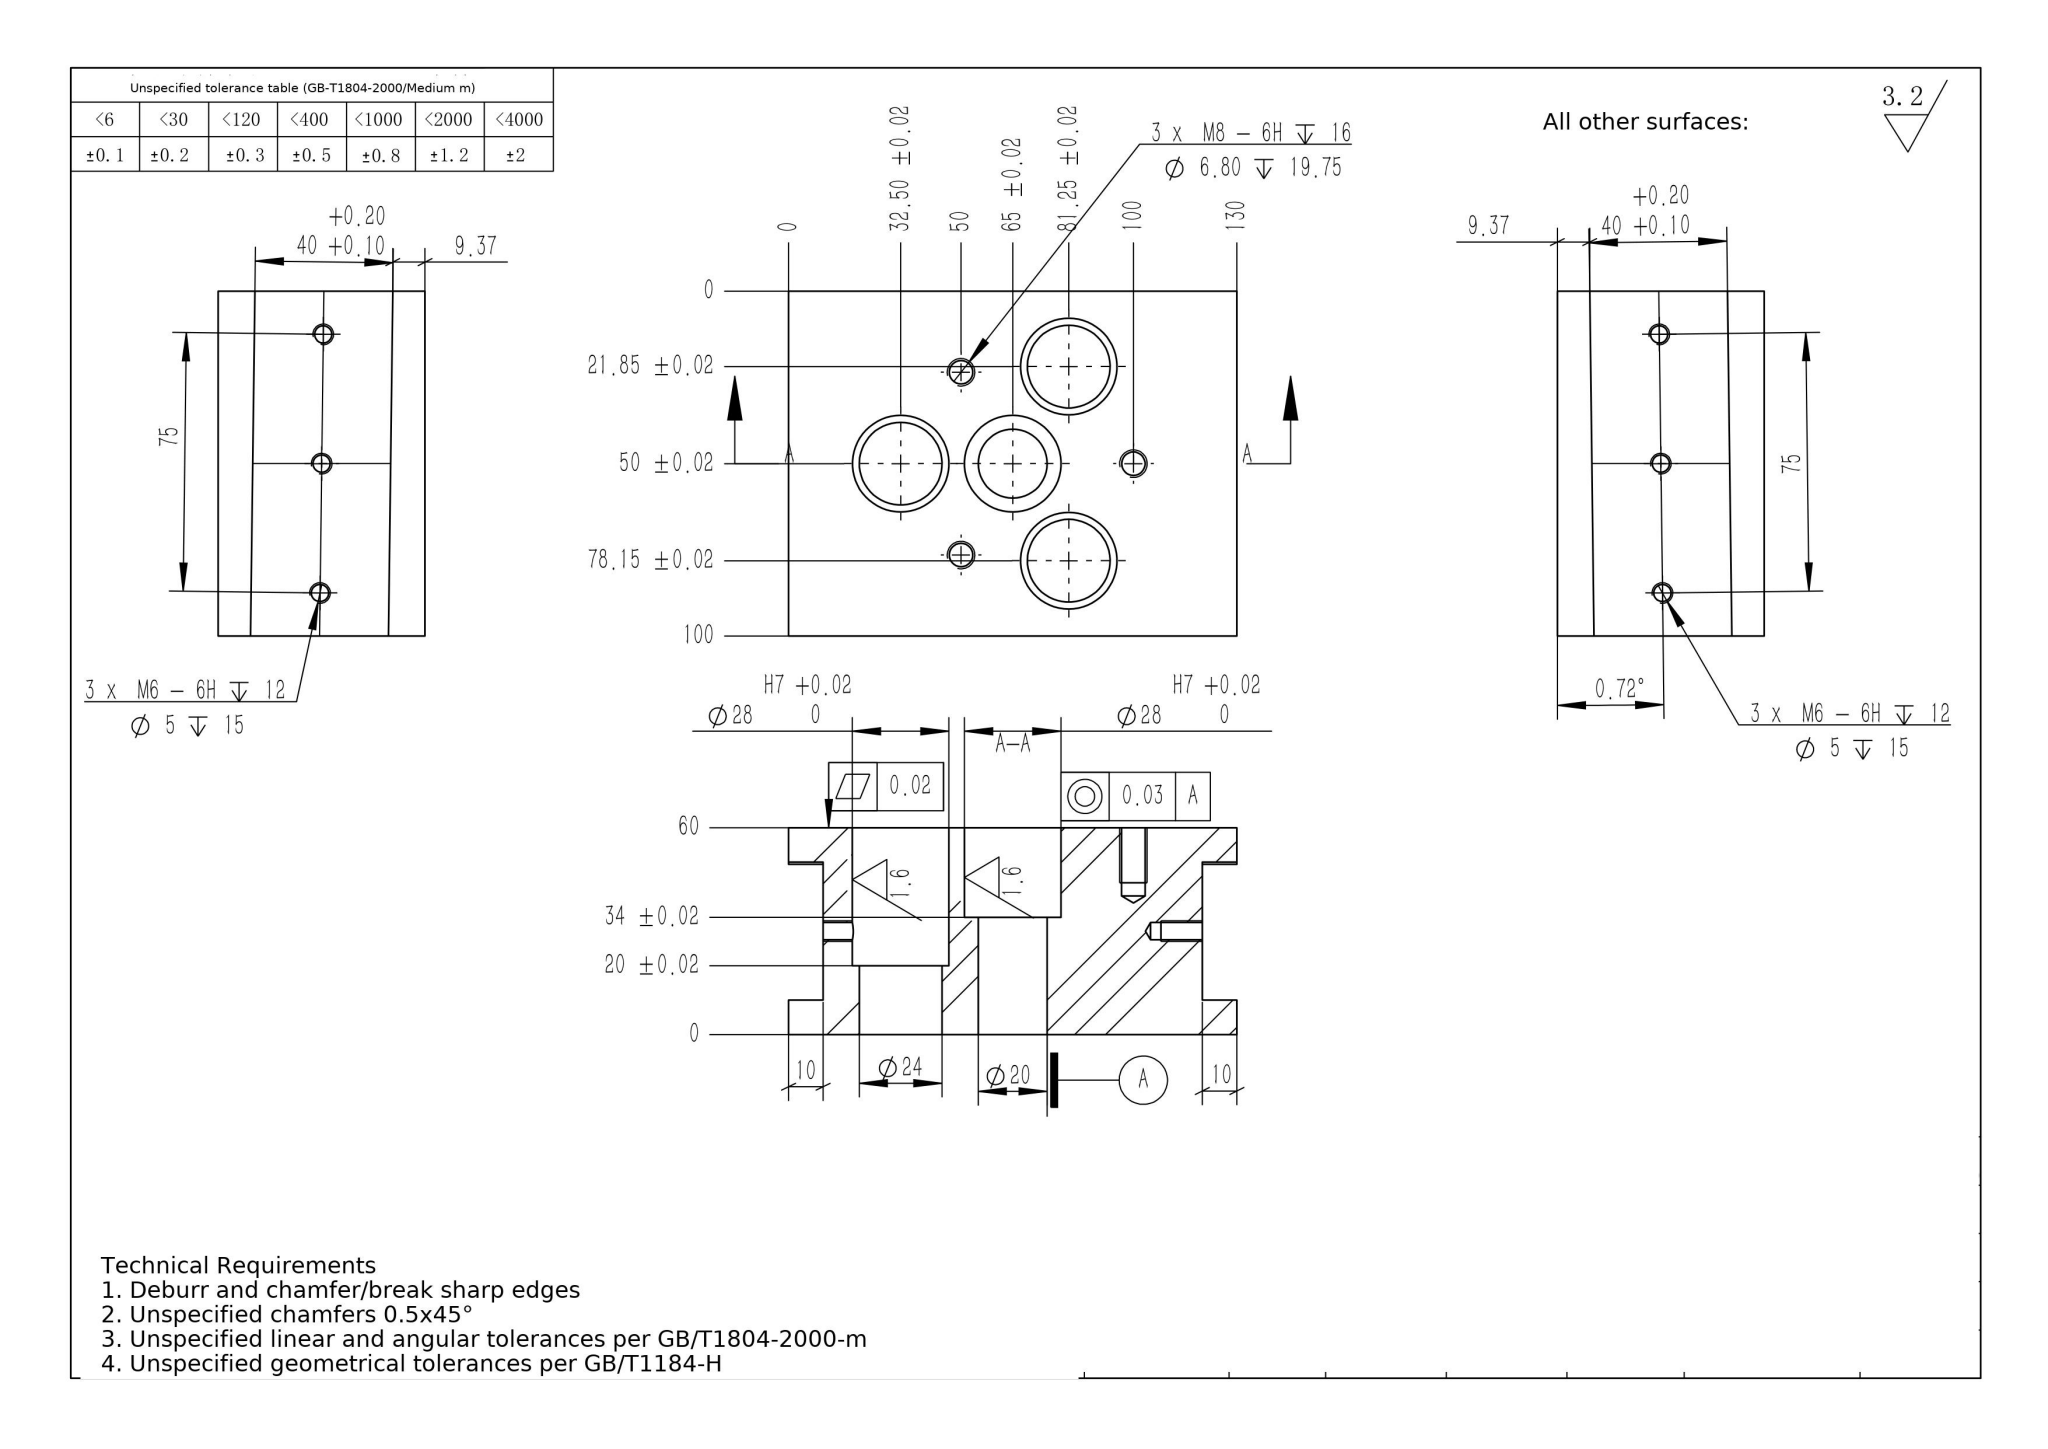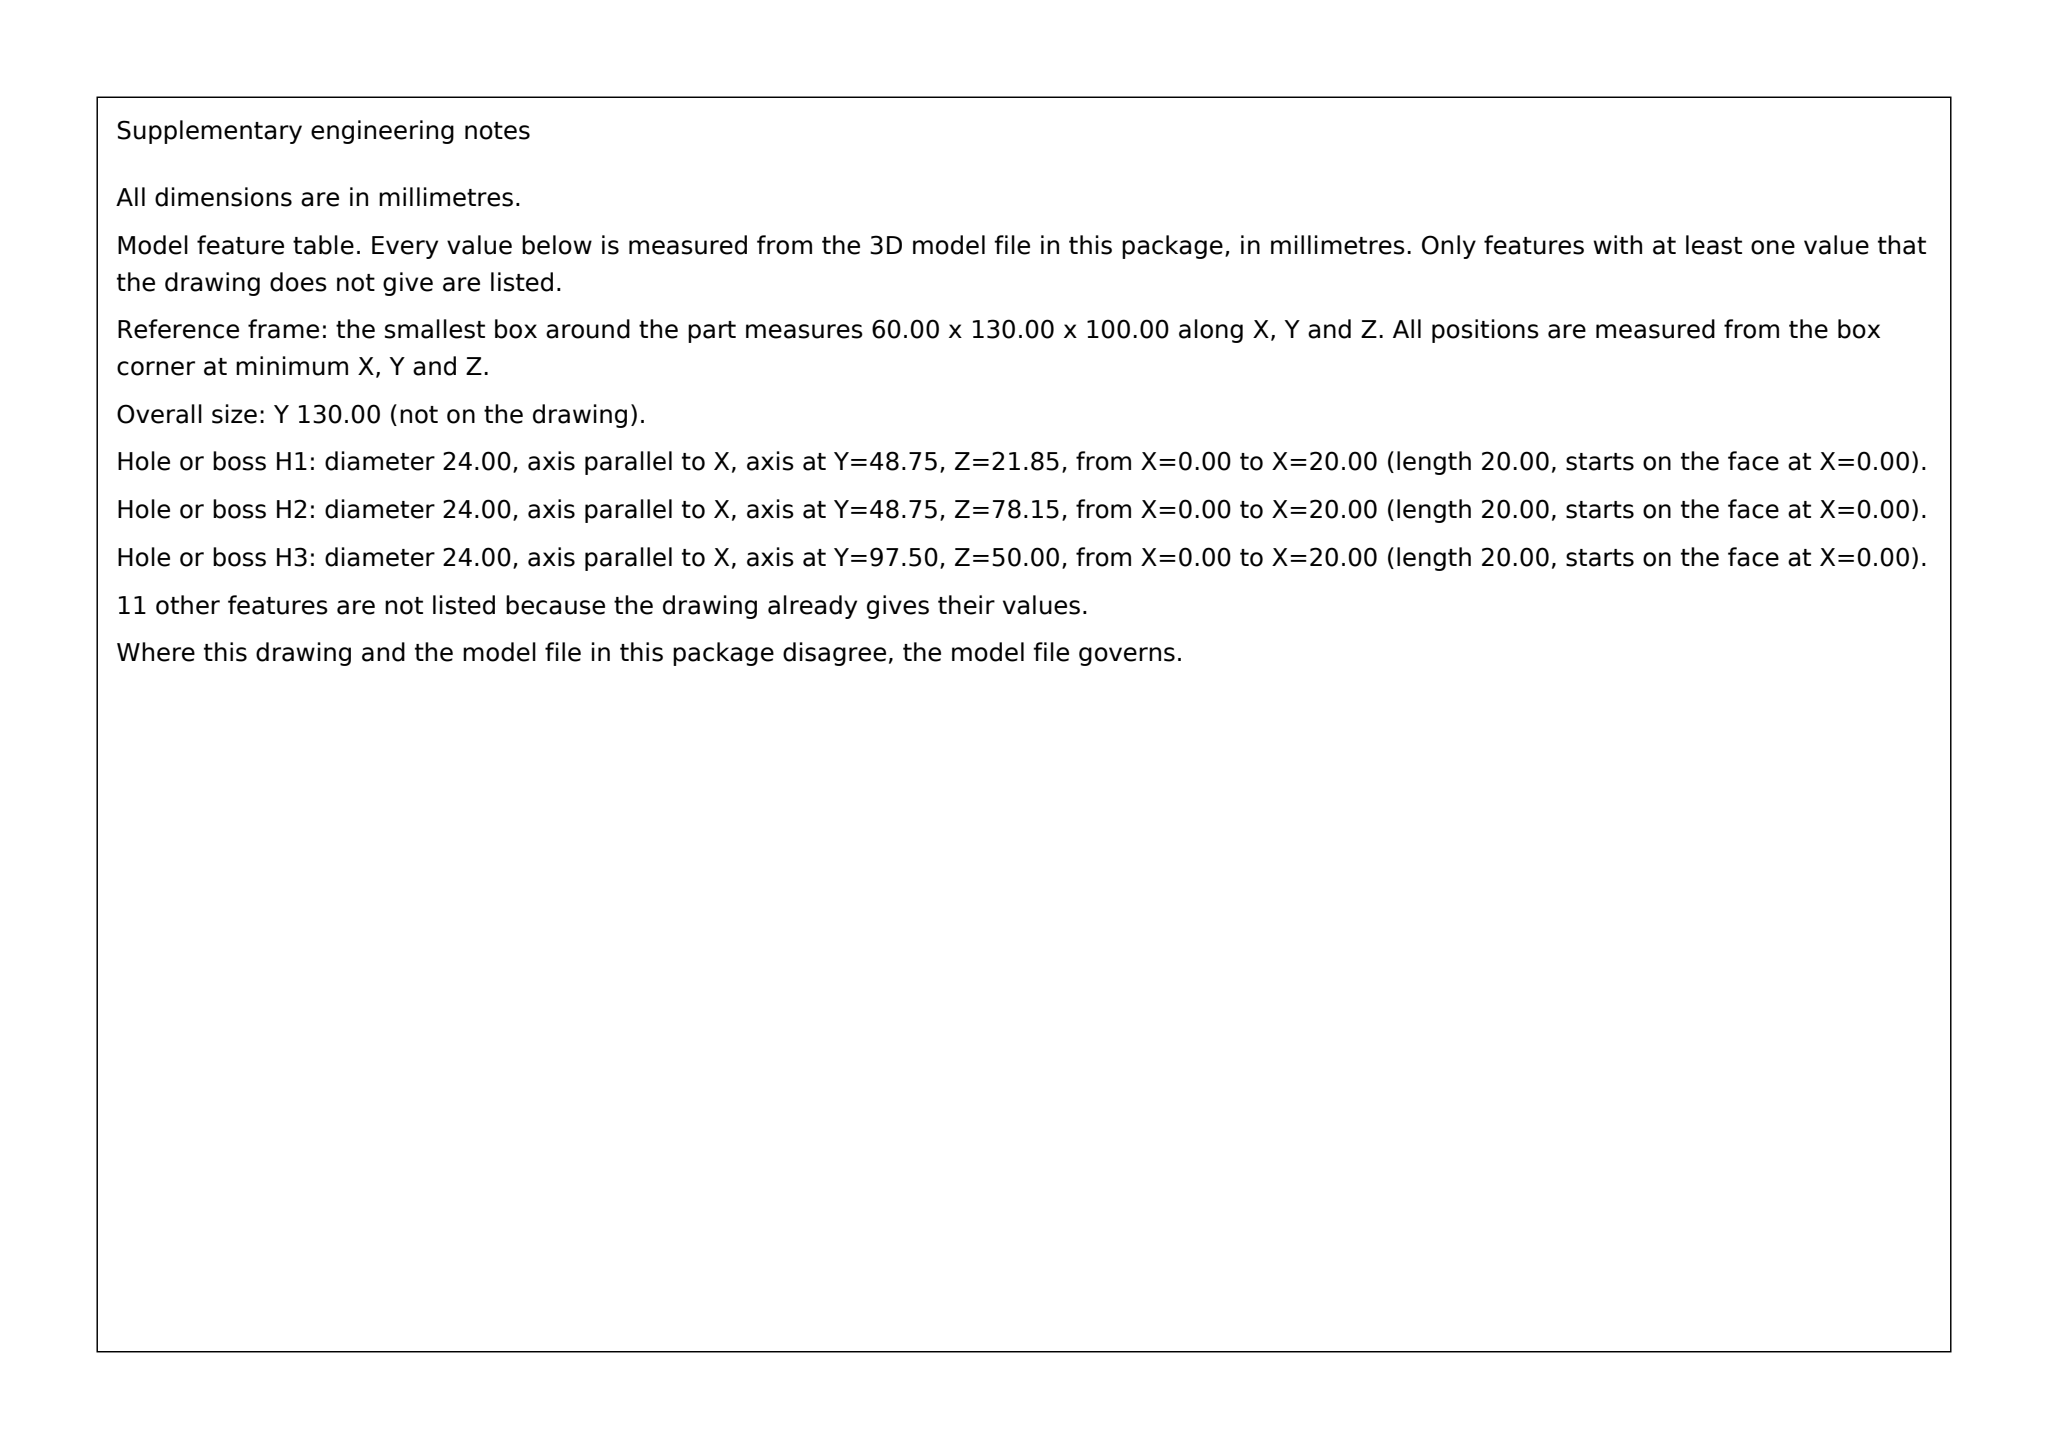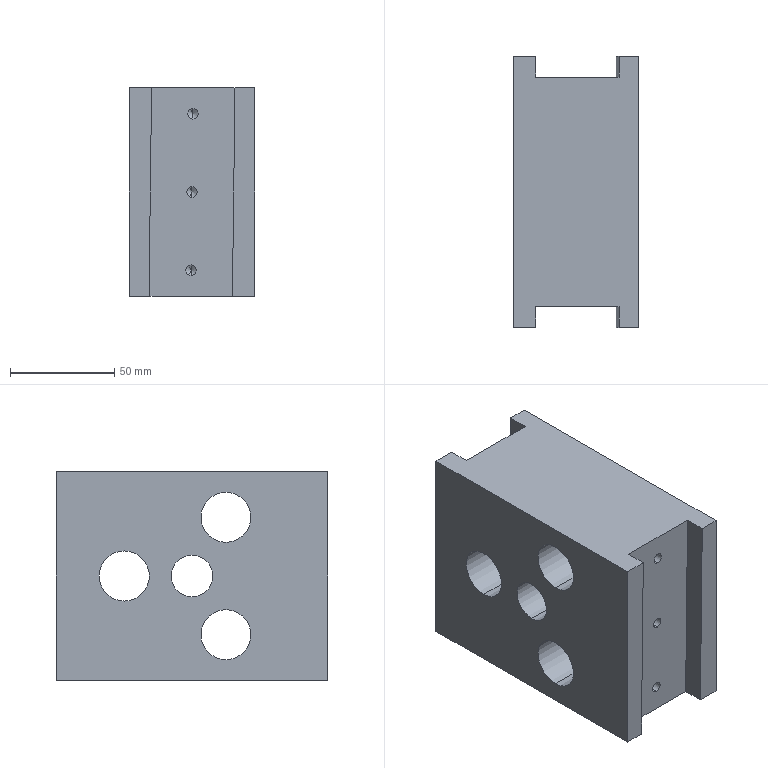Part | SolidWorks | mm | 1 solid | 68 faces | box 60 x 130 x 100 mm | volume 568360 mm3 | cylinder 34 | plane 18 | cone 16 | commonest cylinder face diameters 5 x12 28 x8 6.8 x6 24 x6 20 x2
build123d program:
from build123d import *

# Parameters (mm, degrees)
SKETCH1_W             = 100
SKETCH1_H             = 130
BOSS_EXTRUDE1_DEPTH   = 60
SKETCH2_R             = 14
CUT_EXTRUDE1_DEPTH    = 40
SKETCH3_R             = 14
CUT_EXTRUDE2_DEPTH    = 26
SKETCH4_R             = 10
CUT_EXTRUDE3_DEPTH    = 89.775
SKETCH5_R             = 12
CUT_EXTRUDE4_DEPTH    = 92.241
CUT_EXTRUDE5_DEPTH    = 10
CUT_EXTRUDE6_DEPTH    = 10
M8_TAPPED_HOLE1_D     = 6.8
M8_TAPPED_HOLE1_DEPTH = 19.75
M8_TAPPED_HOLE1_TIP   = 2.043
M6_TAPPED_HOLE1_D     = 5
M6_TAPPED_HOLE1_DEPTH = 15
M6_TAPPED_HOLE1_TIP   = 1.502
M6_TAPPED_HOLE2_D     = 5
M6_TAPPED_HOLE2_DEPTH = 15
M6_TAPPED_HOLE2_TIP   = 1.502


with BuildPart() as part:
    # Sketch1 → Boss-Extrude1 (new body)
    with BuildSketch(Plane(origin=(0, 0, 0), x_dir=(0, 0, -1), z_dir=(1, 0, 0))):
        Rectangle(SKETCH1_W, SKETCH1_H)
    extrude(amount=BOSS_EXTRUDE1_DEPTH)

    # Sketch2 → Cut-Extrude1 (cut)
    with BuildSketch(Plane(origin=(60, 0, 0), x_dir=(0, 0, -1), z_dir=(1, 0, 0))):
        with Locations((0, 32.5)):
            Circle(SKETCH2_R)
        with Locations((28.146, -16.25)):
            Circle(SKETCH2_R)
        with Locations((-28.146, -16.25)):
            Circle(SKETCH2_R)
    extrude(amount=-CUT_EXTRUDE1_DEPTH, mode=Mode.SUBTRACT)

    # Sketch3 → Cut-Extrude2 (cut)
    with BuildSketch(Plane(origin=(60, 0, 0), x_dir=(0, 0, -1), z_dir=(1, 0, 0))):
        Circle(SKETCH3_R)
    extrude(amount=-CUT_EXTRUDE2_DEPTH, mode=Mode.SUBTRACT)

    # Sketch4 → Cut-Extrude3 (cut, through all)
    with BuildSketch(Plane(origin=(34, 0, 0), x_dir=(0, 0, -1), z_dir=(1, 0, 0))):
        Circle(SKETCH4_R)
    extrude(amount=-CUT_EXTRUDE3_DEPTH, mode=Mode.SUBTRACT)

    # Sketch5 → Cut-Extrude4 (cut, through all)
    with BuildSketch(Plane(origin=(20, 0, 0), x_dir=(0, 0, -1), z_dir=(1, 0, 0))):
        with Locations((0, 32.5)):
            Circle(SKETCH5_R)
        with Locations((28.146, -16.25)):
            Circle(SKETCH5_R)
        with Locations((-28.146, -16.25)):
            Circle(SKETCH5_R)
    extrude(amount=-CUT_EXTRUDE4_DEPTH, mode=Mode.SUBTRACT)

    # Sketch8 → Cut-Extrude5 (cut)
    with BuildSketch(Plane(origin=(0, 65, 0), x_dir=(1, 0, 0), z_dir=(0, 1, 0))):
        Polygon((9.373, 50), (10.623, -50), (50.623, -50), (49.373, 50), align=None)
    extrude(amount=-CUT_EXTRUDE5_DEPTH, mode=Mode.SUBTRACT)

    # Sketch9 → Cut-Extrude6 (cut)
    with BuildSketch(Plane.XZ.offset(65)):
        Polygon((10.623, 50), (50.623, 50), (49.373, -50), (9.373, -50), align=None)
    extrude(amount=-CUT_EXTRUDE6_DEPTH, mode=Mode.SUBTRACT)

    # M8 Tapped Hole1
    with Locations(Plane(origin=(60, 0, 0), x_dir=(0, 0, -1), z_dir=(1, 0, 0))):
        with Locations((0, -35), (-26.5, 15), (26.5, 15)):
            Hole(M8_TAPPED_HOLE1_D / 2, depth=M8_TAPPED_HOLE1_DEPTH)
            with Locations((0, 0, -(M8_TAPPED_HOLE1_DEPTH + M8_TAPPED_HOLE1_TIP / 2))):  # 118° drill point
                Cone(0, M8_TAPPED_HOLE1_D / 2, M8_TAPPED_HOLE1_TIP, mode=Mode.SUBTRACT)

    # M6 Tapped Hole1
    with Locations(Plane(origin=(0, -55, 0), x_dir=(-1, 0, 0), z_dir=(0, -1, 0))):
        with Locations((-30.467, -37.497), (-29.998, 0), (-29.53, 37.497)):
            Hole(M6_TAPPED_HOLE1_D / 2, depth=M6_TAPPED_HOLE1_DEPTH)
            with Locations((0, 0, -(M6_TAPPED_HOLE1_DEPTH + M6_TAPPED_HOLE1_TIP / 2))):  # 118° drill point
                Cone(0, M6_TAPPED_HOLE1_D / 2, M6_TAPPED_HOLE1_TIP, mode=Mode.SUBTRACT)

    # M6 Tapped Hole2
    with Locations(Plane(origin=(0, 55, 0), x_dir=(1, 0, 0), z_dir=(0, 1, 0))):
        with Locations((30.467, -37.497), (29.998, 0), (29.53, 37.497)):
            Hole(M6_TAPPED_HOLE2_D / 2, depth=M6_TAPPED_HOLE2_DEPTH)
            with Locations((0, 0, -(M6_TAPPED_HOLE2_DEPTH + M6_TAPPED_HOLE2_TIP / 2))):  # 118° drill point
                Cone(0, M6_TAPPED_HOLE2_D / 2, M6_TAPPED_HOLE2_TIP, mode=Mode.SUBTRACT)


solid = part.part